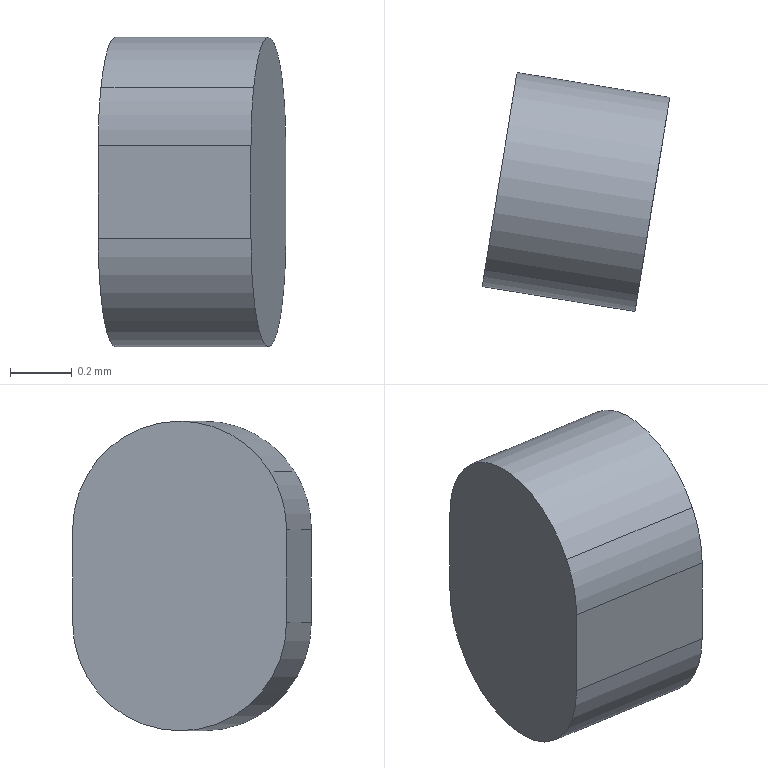Component | SolidWorks | Part30^Assembly1-4 | 1 solid | 7 faces | box 0.61 x 0.77 x 1 mm | volume 0 mm3 | plane 4 | cylinder 3 | commonest cylinder face diameters 0.7 x3
STEP:
#1=COLOUR_RGB('',0.7922,0.8196,0.9333);
#2=FILL_AREA_STYLE_COLOUR('',#1);
#3=FILL_AREA_STYLE('',(#2));
#4=SURFACE_STYLE_FILL_AREA(#3);
#5=SURFACE_SIDE_STYLE('',(#4));
#6=SURFACE_STYLE_USAGE(.BOTH.,#5);
#7=PRESENTATION_STYLE_ASSIGNMENT((#6));
#8=CARTESIAN_POINT('',(0.5388,-0.1572,0.1905));
#9=VERTEX_POINT('',#8);
#10=CARTESIAN_POINT('',(0.5385,-0.1593,0.1831));
#11=VERTEX_POINT('',#10);
#12=CARTESIAN_POINT('',(0.5407,-0.1457,0.1831));
#13=DIRECTION('',(0.987,-0.1605,-0.));
#14=DIRECTION('',(0.1355,0.8335,-0.5357));
#15=AXIS2_PLACEMENT_3D('',#12,#13,#14);
#16=CIRCLE('',#15,0.01378);
#17=EDGE_CURVE('',#9,#11,#16,.T.);
#18=ORIENTED_EDGE('',*,*,#17,.F.);
#19=CARTESIAN_POINT('',(0.5194,-0.154,0.1905));
#20=VERTEX_POINT('',#19);
#21=CARTESIAN_POINT('',(0.5388,-0.1572,0.1905));
#22=DIRECTION('',(-0.987,0.1605,0.));
#23=VECTOR('',#22,39.37);
#24=LINE('',#21,#23);
#25=EDGE_CURVE('',#9,#20,#24,.T.);
#26=ORIENTED_EDGE('',*,*,#25,.T.);
#27=CARTESIAN_POINT('',(0.5191,-0.1561,0.1831));
#28=VERTEX_POINT('',#27);
#29=CARTESIAN_POINT('',(0.5213,-0.1425,0.1831));
#30=DIRECTION('',(0.987,-0.1605,-0.));
#31=DIRECTION('',(0.1355,0.8335,-0.5357));
#32=AXIS2_PLACEMENT_3D('',#29,#30,#31);
#33=CIRCLE('',#32,0.01378);
#34=EDGE_CURVE('',#20,#28,#33,.T.);
#35=ORIENTED_EDGE('',*,*,#34,.T.);
#36=CARTESIAN_POINT('',(0.5385,-0.1593,0.1831));
#37=DIRECTION('',(-0.987,0.1605,0.));
#38=VECTOR('',#37,39.37);
#39=LINE('',#36,#38);
#40=EDGE_CURVE('',#11,#28,#39,.T.);
#41=ORIENTED_EDGE('',*,*,#40,.F.);
#42=EDGE_LOOP('',(#18,#26,#35,#41));
#43=FACE_OUTER_BOUND('',#42,.T.);
#44=CARTESIAN_POINT('',(0.5407,-0.1457,0.1831));
#45=DIRECTION('',(-0.987,0.1605,0.));
#46=DIRECTION('',(-0.1355,-0.8335,0.5357));
#47=AXIS2_PLACEMENT_3D('',#44,#45,#46);
#48=CYLINDRICAL_SURFACE('',#47,0.01378);
#49=ADVANCED_FACE('',(#43),#48,.T.);
#50=ORIENTED_EDGE('',*,*,#25,.F.);
#51=CARTESIAN_POINT('',(0.5429,-0.1321,0.1831));
#52=VERTEX_POINT('',#51);
#53=CARTESIAN_POINT('',(0.5407,-0.1457,0.1831));
#54=DIRECTION('',(0.987,-0.1605,-0.));
#55=DIRECTION('',(0.1355,0.8335,-0.5357));
#56=AXIS2_PLACEMENT_3D('',#53,#54,#55);
#57=CIRCLE('',#56,0.01378);
#58=EDGE_CURVE('',#52,#9,#57,.T.);
#59=ORIENTED_EDGE('',*,*,#58,.F.);
#60=CARTESIAN_POINT('',(0.5235,-0.1289,0.1831));
#61=VERTEX_POINT('',#60);
#62=CARTESIAN_POINT('',(0.5429,-0.1321,0.1831));
#63=DIRECTION('',(-0.987,0.1605,0.));
#64=VECTOR('',#63,39.37);
#65=LINE('',#62,#64);
#66=EDGE_CURVE('',#52,#61,#65,.T.);
#67=ORIENTED_EDGE('',*,*,#66,.T.);
#68=CARTESIAN_POINT('',(0.5213,-0.1425,0.1831));
#69=DIRECTION('',(0.987,-0.1605,-0.));
#70=DIRECTION('',(0.1355,0.8335,-0.5357));
#71=AXIS2_PLACEMENT_3D('',#68,#69,#70);
#72=CIRCLE('',#71,0.01378);
#73=EDGE_CURVE('',#61,#20,#72,.T.);
#74=ORIENTED_EDGE('',*,*,#73,.T.);
#75=EDGE_LOOP('',(#50,#59,#67,#74));
#76=FACE_OUTER_BOUND('',#75,.T.);
#77=CARTESIAN_POINT('',(0.5407,-0.1457,0.1831));
#78=DIRECTION('',(-0.987,0.1605,0.));
#79=DIRECTION('',(-0.1355,-0.8335,0.5357));
#80=AXIS2_PLACEMENT_3D('',#77,#78,#79);
#81=CYLINDRICAL_SURFACE('',#80,0.01378);
#82=ADVANCED_FACE('',(#76),#81,.T.);
#83=CARTESIAN_POINT('',(0.5191,-0.1561,0.1713));
#84=VERTEX_POINT('',#83);
#85=CARTESIAN_POINT('',(0.5191,-0.1561,0.1831));
#86=DIRECTION('',(-0.,-0.,-1.));
#87=VECTOR('',#86,39.37);
#88=LINE('',#85,#87);
#89=EDGE_CURVE('',#28,#84,#88,.T.);
#90=ORIENTED_EDGE('',*,*,#89,.T.);
#91=CARTESIAN_POINT('',(0.5385,-0.1593,0.1713));
#92=VERTEX_POINT('',#91);
#93=CARTESIAN_POINT('',(0.5385,-0.1593,0.1713));
#94=DIRECTION('',(-0.987,0.1605,0.));
#95=VECTOR('',#94,39.37);
#96=LINE('',#93,#95);
#97=EDGE_CURVE('',#92,#84,#96,.T.);
#98=ORIENTED_EDGE('',*,*,#97,.F.);
#99=CARTESIAN_POINT('',(0.5385,-0.1593,0.1831));
#100=DIRECTION('',(-0.,-0.,-1.));
#101=VECTOR('',#100,39.37);
#102=LINE('',#99,#101);
#103=EDGE_CURVE('',#11,#92,#102,.T.);
#104=ORIENTED_EDGE('',*,*,#103,.F.);
#105=ORIENTED_EDGE('',*,*,#40,.T.);
#106=EDGE_LOOP('',(#90,#98,#104,#105));
#107=FACE_OUTER_BOUND('',#106,.T.);
#108=CARTESIAN_POINT('',(0.5385,-0.1593,0.1831));
#109=DIRECTION('',(0.1605,0.987,0.));
#110=DIRECTION('',(0.,-0.,1.));
#111=AXIS2_PLACEMENT_3D('',#108,#109,#110);
#112=PLANE('',#111);
#113=ADVANCED_FACE('',(#107),#112,.F.);
#114=CARTESIAN_POINT('',(0.5235,-0.1289,0.1713));
#115=VERTEX_POINT('',#114);
#116=CARTESIAN_POINT('',(0.5213,-0.1425,0.1713));
#117=DIRECTION('',(0.987,-0.1605,-0.));
#118=DIRECTION('',(0.1355,0.8335,-0.5357));
#119=AXIS2_PLACEMENT_3D('',#116,#117,#118);
#120=CIRCLE('',#119,0.01378);
#121=EDGE_CURVE('',#84,#115,#120,.T.);
#122=ORIENTED_EDGE('',*,*,#121,.T.);
#123=CARTESIAN_POINT('',(0.5429,-0.1321,0.1713));
#124=VERTEX_POINT('',#123);
#125=CARTESIAN_POINT('',(0.5429,-0.1321,0.1713));
#126=DIRECTION('',(-0.987,0.1605,0.));
#127=VECTOR('',#126,39.37);
#128=LINE('',#125,#127);
#129=EDGE_CURVE('',#124,#115,#128,.T.);
#130=ORIENTED_EDGE('',*,*,#129,.F.);
#131=CARTESIAN_POINT('',(0.5407,-0.1457,0.1713));
#132=DIRECTION('',(0.987,-0.1605,-0.));
#133=DIRECTION('',(0.1355,0.8335,-0.5357));
#134=AXIS2_PLACEMENT_3D('',#131,#132,#133);
#135=CIRCLE('',#134,0.01378);
#136=EDGE_CURVE('',#92,#124,#135,.T.);
#137=ORIENTED_EDGE('',*,*,#136,.F.);
#138=ORIENTED_EDGE('',*,*,#97,.T.);
#139=EDGE_LOOP('',(#122,#130,#137,#138));
#140=FACE_OUTER_BOUND('',#139,.T.);
#141=CARTESIAN_POINT('',(0.5407,-0.1457,0.1713));
#142=DIRECTION('',(-0.987,0.1605,0.));
#143=DIRECTION('',(-0.1355,-0.8335,0.5357));
#144=AXIS2_PLACEMENT_3D('',#141,#142,#143);
#145=CYLINDRICAL_SURFACE('',#144,0.01378);
#146=ADVANCED_FACE('',(#140),#145,.T.);
#147=CARTESIAN_POINT('',(0.5235,-0.1289,0.1831));
#148=DIRECTION('',(0.,0.,1.));
#149=VECTOR('',#148,39.37);
#150=LINE('',#147,#149);
#151=EDGE_CURVE('',#115,#61,#150,.T.);
#152=ORIENTED_EDGE('',*,*,#151,.T.);
#153=ORIENTED_EDGE('',*,*,#66,.F.);
#154=CARTESIAN_POINT('',(0.5429,-0.1321,0.1831));
#155=DIRECTION('',(0.,0.,1.));
#156=VECTOR('',#155,39.37);
#157=LINE('',#154,#156);
#158=EDGE_CURVE('',#124,#52,#157,.T.);
#159=ORIENTED_EDGE('',*,*,#158,.F.);
#160=ORIENTED_EDGE('',*,*,#129,.T.);
#161=EDGE_LOOP('',(#152,#153,#159,#160));
#162=FACE_OUTER_BOUND('',#161,.T.);
#163=CARTESIAN_POINT('',(0.5429,-0.1321,0.1831));
#164=DIRECTION('',(-0.1605,-0.987,0.));
#165=DIRECTION('',(-0.,-0.,-1.));
#166=AXIS2_PLACEMENT_3D('',#163,#164,#165);
#167=PLANE('',#166);
#168=ADVANCED_FACE('',(#162),#167,.F.);
#169=ORIENTED_EDGE('',*,*,#58,.T.);
#170=ORIENTED_EDGE('',*,*,#17,.T.);
#171=ORIENTED_EDGE('',*,*,#103,.T.);
#172=ORIENTED_EDGE('',*,*,#136,.T.);
#173=ORIENTED_EDGE('',*,*,#158,.T.);
#174=EDGE_LOOP('',(#169,#170,#171,#172,#173));
#175=FACE_OUTER_BOUND('',#174,.T.);
#176=CARTESIAN_POINT('',(0.5407,-0.1457,0.1831));
#177=DIRECTION('',(0.987,-0.1605,-0.));
#178=DIRECTION('',(0.1355,0.8335,-0.5357));
#179=AXIS2_PLACEMENT_3D('',#176,#177,#178);
#180=PLANE('',#179);
#181=ADVANCED_FACE('',(#175),#180,.T.);
#182=ORIENTED_EDGE('',*,*,#73,.F.);
#183=ORIENTED_EDGE('',*,*,#151,.F.);
#184=ORIENTED_EDGE('',*,*,#121,.F.);
#185=ORIENTED_EDGE('',*,*,#89,.F.);
#186=ORIENTED_EDGE('',*,*,#34,.F.);
#187=EDGE_LOOP('',(#182,#183,#184,#185,#186));
#188=FACE_OUTER_BOUND('',#187,.T.);
#189=CARTESIAN_POINT('',(0.5213,-0.1425,0.1831));
#190=DIRECTION('',(0.987,-0.1605,-0.));
#191=DIRECTION('',(0.1355,0.8335,-0.5357));
#192=AXIS2_PLACEMENT_3D('',#189,#190,#191);
#193=PLANE('',#192);
#194=ADVANCED_FACE('',(#188),#193,.F.);
#195=CLOSED_SHELL('',(#49,#82,#113,#146,#168,#181,#194));
#196=MANIFOLD_SOLID_BREP('',#195);
#197=STYLED_ITEM('',(#7),#196);
#198=PRESENTATION_LAYER_ASSIGNMENT('','',(#197));
#199=(LENGTH_UNIT()NAMED_UNIT(*)SI_UNIT($,.METRE.));
#200=LENGTH_MEASURE_WITH_UNIT(LENGTH_MEASURE(0.0254),#199);
#201=DIMENSIONAL_EXPONENTS(1.,0.,0.,0.,0.,0.,0.);
#202=(CONVERSION_BASED_UNIT('',#200)LENGTH_UNIT()NAMED_UNIT(#201));
#203=UNCERTAINTY_MEASURE_WITH_UNIT(LENGTH_MEASURE(0.00001),#202,'','');
#204=(NAMED_UNIT(*)PLANE_ANGLE_UNIT()SI_UNIT($,.RADIAN.));
#205=(NAMED_UNIT(*)SI_UNIT($,.STERADIAN.)SOLID_ANGLE_UNIT());
#206=(GEOMETRIC_REPRESENTATION_CONTEXT(3)GLOBAL_UNCERTAINTY_ASSIGNED_CONTEXT((#203))GLOBAL_UNIT_ASSIGNED_CONTEXT((#202,#204,#205))REPRESENTATION_CONTEXT('',''));
#207=MECHANICAL_DESIGN_GEOMETRIC_PRESENTATION_REPRESENTATION('',(#197),#206);
#208=CARTESIAN_POINT('',(0.,0.,0.));
#209=DIRECTION('',(0.,0.,1.));
#210=DIRECTION('',(1.,0.,0.));
#211=AXIS2_PLACEMENT_3D('',#208,#209,#210);
#212=(LENGTH_UNIT()NAMED_UNIT(*)SI_UNIT($,.METRE.));
#213=LENGTH_MEASURE_WITH_UNIT(LENGTH_MEASURE(0.0254),#212);
#214=DIMENSIONAL_EXPONENTS(1.,0.,0.,0.,0.,0.,0.);
#215=(CONVERSION_BASED_UNIT('',#213)LENGTH_UNIT()NAMED_UNIT(#214));
#216=UNCERTAINTY_MEASURE_WITH_UNIT(LENGTH_MEASURE(0.00001),#215,'','');
#217=(NAMED_UNIT(*)PLANE_ANGLE_UNIT()SI_UNIT($,.RADIAN.));
#218=(NAMED_UNIT(*)SI_UNIT($,.STERADIAN.)SOLID_ANGLE_UNIT());
#219=(GEOMETRIC_REPRESENTATION_CONTEXT(3)GLOBAL_UNCERTAINTY_ASSIGNED_CONTEXT((#216))GLOBAL_UNIT_ASSIGNED_CONTEXT((#215,#217,#218))REPRESENTATION_CONTEXT('',''));
#220=ADVANCED_BREP_SHAPE_REPRESENTATION('',(#196,#211),#219);